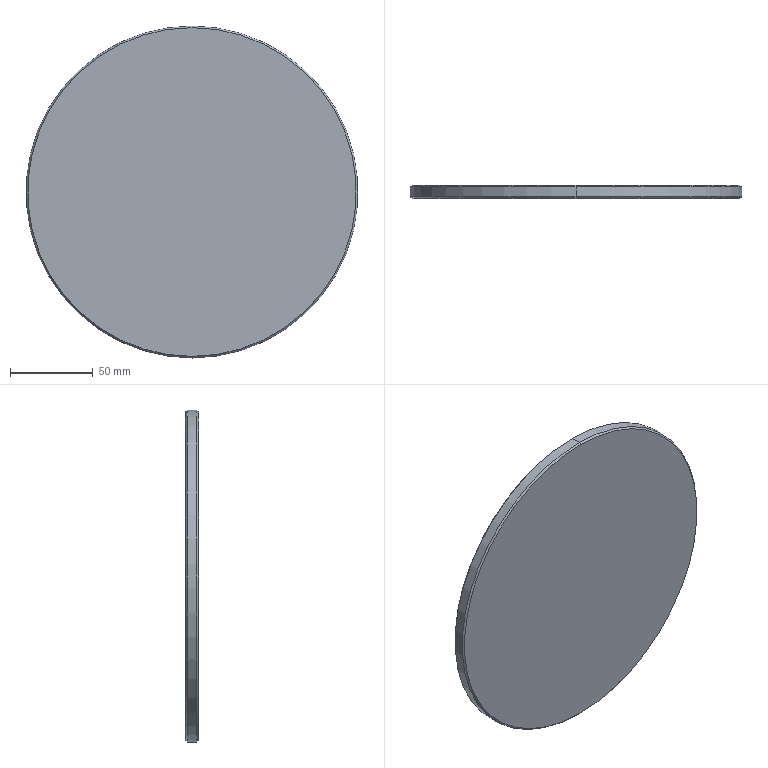Component | SolidWorks | Inline-H010-H01-001K-1 | 1 solid | 8 faces | box 200 x 8 x 200 mm | volume 250701 mm3 | cone 4 | cylinder 2 | plane 2 | commonest cylinder face diameters 200 x2
build123d program:
from build123d import *

# Parameters (mm, degrees)
SKETCH1_R           = 100
BOSS_EXTRUDE1_DEPTH = 4
CHAMFER1_SIZE       = 1


with BuildPart() as part:
    # Sketch1 → Boss-Extrude1 (new, symmetric)
    with BuildSketch(Plane.XY):
        Circle(SKETCH1_R)
    extrude(amount=BOSS_EXTRUDE1_DEPTH, both=True)

    # Chamfer1
    chamfer1_edges = [part.edges().sort_by_distance(p)[0] for p in [
        (-100, 0, -4),
        (-100, 0, 4),
    ]]
    chamfer(chamfer1_edges, length=CHAMFER1_SIZE)


solid = part.part

# Placed as in the assembly
solid = solid.moved(Location((29.082, -10.032, 139.665), (90, 0, 0)))
STEP:
#1=CARTESIAN_POINT('',(1.145,-0.2375,9.396));
#2=VERTEX_POINT('',#1);
#3=CARTESIAN_POINT('',(1.145,-0.2375,1.601));
#4=VERTEX_POINT('',#3);
#5=CARTESIAN_POINT('',(1.145,-0.2375,5.499));
#6=DIRECTION('',(-0.,1.,0.));
#7=DIRECTION('',(0.,0.,-1.));
#8=AXIS2_PLACEMENT_3D('',#5,#6,#7);
#9=CIRCLE('',#8,3.898);
#10=EDGE_CURVE('',#2,#4,#9,.T.);
#11=ORIENTED_EDGE('',*,*,#10,.F.);
#12=CARTESIAN_POINT('',(1.145,-0.2769,9.436));
#13=VERTEX_POINT('',#12);
#14=CARTESIAN_POINT('',(1.145,-0.2769,9.436));
#15=DIRECTION('',(0.,-0.7071,0.7071));
#16=VECTOR('',#15,39.37);
#17=LINE('',#14,#16);
#18=EDGE_CURVE('',#2,#13,#17,.T.);
#19=ORIENTED_EDGE('',*,*,#18,.T.);
#20=CARTESIAN_POINT('',(1.145,-0.2769,1.562));
#21=VERTEX_POINT('',#20);
#22=CARTESIAN_POINT('',(1.145,-0.2769,5.499));
#23=DIRECTION('',(0.,-1.,-0.));
#24=DIRECTION('',(0.,0.,-1.));
#25=AXIS2_PLACEMENT_3D('',#22,#23,#24);
#26=CIRCLE('',#25,3.937);
#27=EDGE_CURVE('',#21,#13,#26,.T.);
#28=ORIENTED_EDGE('',*,*,#27,.F.);
#29=CARTESIAN_POINT('',(1.145,-0.2769,1.562));
#30=DIRECTION('',(0.,-0.7071,-0.7071));
#31=VECTOR('',#30,39.37);
#32=LINE('',#29,#31);
#33=EDGE_CURVE('',#4,#21,#32,.T.);
#34=ORIENTED_EDGE('',*,*,#33,.F.);
#35=EDGE_LOOP('',(#11,#19,#28,#34));
#36=FACE_OUTER_BOUND('',#35,.T.);
#37=CARTESIAN_POINT('',(1.145,-0.2769,5.499));
#38=DIRECTION('',(0.,-1.,-0.));
#39=DIRECTION('',(0.,0.,-1.));
#40=AXIS2_PLACEMENT_3D('',#37,#38,#39);
#41=CONICAL_SURFACE('',#40,3.937,0.7854);
#42=ADVANCED_FACE('',(#36),#41,.T.);
#43=CARTESIAN_POINT('',(1.145,-0.5525,1.601));
#44=VERTEX_POINT('',#43);
#45=CARTESIAN_POINT('',(1.145,-0.5525,9.396));
#46=VERTEX_POINT('',#45);
#47=CARTESIAN_POINT('',(1.145,-0.5525,5.499));
#48=DIRECTION('',(0.,-1.,-0.));
#49=DIRECTION('',(0.,0.,-1.));
#50=AXIS2_PLACEMENT_3D('',#47,#48,#49);
#51=CIRCLE('',#50,3.898);
#52=EDGE_CURVE('',#44,#46,#51,.T.);
#53=ORIENTED_EDGE('',*,*,#52,.F.);
#54=CARTESIAN_POINT('',(1.145,-0.5131,1.562));
#55=VERTEX_POINT('',#54);
#56=CARTESIAN_POINT('',(1.145,-0.5525,1.601));
#57=DIRECTION('',(0.,0.7071,-0.7071));
#58=VECTOR('',#57,39.37);
#59=LINE('',#56,#58);
#60=EDGE_CURVE('',#44,#55,#59,.T.);
#61=ORIENTED_EDGE('',*,*,#60,.T.);
#62=CARTESIAN_POINT('',(1.145,-0.5131,9.436));
#63=VERTEX_POINT('',#62);
#64=CARTESIAN_POINT('',(1.145,-0.5131,5.499));
#65=DIRECTION('',(-0.,1.,0.));
#66=DIRECTION('',(0.,0.,-1.));
#67=AXIS2_PLACEMENT_3D('',#64,#65,#66);
#68=CIRCLE('',#67,3.937);
#69=EDGE_CURVE('',#63,#55,#68,.T.);
#70=ORIENTED_EDGE('',*,*,#69,.F.);
#71=CARTESIAN_POINT('',(1.145,-0.5525,9.396));
#72=DIRECTION('',(-0.,0.7071,0.7071));
#73=VECTOR('',#72,39.37);
#74=LINE('',#71,#73);
#75=EDGE_CURVE('',#46,#63,#74,.T.);
#76=ORIENTED_EDGE('',*,*,#75,.F.);
#77=EDGE_LOOP('',(#53,#61,#70,#76));
#78=FACE_OUTER_BOUND('',#77,.T.);
#79=CARTESIAN_POINT('',(1.145,-0.5525,5.499));
#80=DIRECTION('',(-0.,1.,0.));
#81=DIRECTION('',(0.,-0.,1.));
#82=AXIS2_PLACEMENT_3D('',#79,#80,#81);
#83=CONICAL_SURFACE('',#82,3.898,0.7854);
#84=ADVANCED_FACE('',(#78),#83,.T.);
#85=ORIENTED_EDGE('',*,*,#69,.T.);
#86=CARTESIAN_POINT('',(1.145,-0.5525,1.562));
#87=DIRECTION('',(-0.,1.,0.));
#88=VECTOR('',#87,39.37);
#89=LINE('',#86,#88);
#90=EDGE_CURVE('',#55,#21,#89,.T.);
#91=ORIENTED_EDGE('',*,*,#90,.T.);
#92=ORIENTED_EDGE('',*,*,#27,.T.);
#93=CARTESIAN_POINT('',(1.145,-0.5525,9.436));
#94=DIRECTION('',(-0.,1.,0.));
#95=VECTOR('',#94,39.37);
#96=LINE('',#93,#95);
#97=EDGE_CURVE('',#63,#13,#96,.T.);
#98=ORIENTED_EDGE('',*,*,#97,.F.);
#99=EDGE_LOOP('',(#85,#91,#92,#98));
#100=FACE_OUTER_BOUND('',#99,.T.);
#101=CARTESIAN_POINT('',(1.145,-0.5525,5.499));
#102=DIRECTION('',(-0.,1.,0.));
#103=DIRECTION('',(0.,-0.,1.));
#104=AXIS2_PLACEMENT_3D('',#101,#102,#103);
#105=CYLINDRICAL_SURFACE('',#104,3.937);
#106=ADVANCED_FACE('',(#100),#105,.T.);
#107=ORIENTED_EDGE('',*,*,#90,.F.);
#108=CARTESIAN_POINT('',(1.145,-0.5131,5.499));
#109=DIRECTION('',(-0.,1.,0.));
#110=DIRECTION('',(0.,0.,-1.));
#111=AXIS2_PLACEMENT_3D('',#108,#109,#110);
#112=CIRCLE('',#111,3.937);
#113=EDGE_CURVE('',#55,#63,#112,.T.);
#114=ORIENTED_EDGE('',*,*,#113,.T.);
#115=ORIENTED_EDGE('',*,*,#97,.T.);
#116=CARTESIAN_POINT('',(1.145,-0.2769,5.499));
#117=DIRECTION('',(0.,-1.,-0.));
#118=DIRECTION('',(0.,0.,-1.));
#119=AXIS2_PLACEMENT_3D('',#116,#117,#118);
#120=CIRCLE('',#119,3.937);
#121=EDGE_CURVE('',#13,#21,#120,.T.);
#122=ORIENTED_EDGE('',*,*,#121,.T.);
#123=EDGE_LOOP('',(#107,#114,#115,#122));
#124=FACE_OUTER_BOUND('',#123,.T.);
#125=CARTESIAN_POINT('',(1.145,-0.5525,5.499));
#126=DIRECTION('',(-0.,1.,0.));
#127=DIRECTION('',(0.,-0.,1.));
#128=AXIS2_PLACEMENT_3D('',#125,#126,#127);
#129=CYLINDRICAL_SURFACE('',#128,3.937);
#130=ADVANCED_FACE('',(#124),#129,.T.);
#131=CARTESIAN_POINT('',(1.145,-0.5525,5.499));
#132=DIRECTION('',(0.,-1.,-0.));
#133=DIRECTION('',(0.,0.,-1.));
#134=AXIS2_PLACEMENT_3D('',#131,#132,#133);
#135=CIRCLE('',#134,3.898);
#136=EDGE_CURVE('',#46,#44,#135,.T.);
#137=ORIENTED_EDGE('',*,*,#136,.T.);
#138=ORIENTED_EDGE('',*,*,#52,.T.);
#139=EDGE_LOOP('',(#137,#138));
#140=FACE_OUTER_BOUND('',#139,.T.);
#141=CARTESIAN_POINT('',(1.145,-0.5525,5.499));
#142=DIRECTION('',(0.,-1.,-0.));
#143=DIRECTION('',(0.,0.,-1.));
#144=AXIS2_PLACEMENT_3D('',#141,#142,#143);
#145=PLANE('',#144);
#146=ADVANCED_FACE('',(#140),#145,.T.);
#147=CARTESIAN_POINT('',(1.145,-0.2375,5.499));
#148=DIRECTION('',(-0.,1.,0.));
#149=DIRECTION('',(0.,0.,-1.));
#150=AXIS2_PLACEMENT_3D('',#147,#148,#149);
#151=CIRCLE('',#150,3.898);
#152=EDGE_CURVE('',#4,#2,#151,.T.);
#153=ORIENTED_EDGE('',*,*,#152,.T.);
#154=ORIENTED_EDGE('',*,*,#10,.T.);
#155=EDGE_LOOP('',(#153,#154));
#156=FACE_OUTER_BOUND('',#155,.T.);
#157=CARTESIAN_POINT('',(1.145,-0.2375,5.499));
#158=DIRECTION('',(0.,-1.,-0.));
#159=DIRECTION('',(0.,0.,-1.));
#160=AXIS2_PLACEMENT_3D('',#157,#158,#159);
#161=PLANE('',#160);
#162=ADVANCED_FACE('',(#156),#161,.F.);
#163=ORIENTED_EDGE('',*,*,#60,.F.);
#164=ORIENTED_EDGE('',*,*,#136,.F.);
#165=ORIENTED_EDGE('',*,*,#75,.T.);
#166=ORIENTED_EDGE('',*,*,#113,.F.);
#167=EDGE_LOOP('',(#163,#164,#165,#166));
#168=FACE_OUTER_BOUND('',#167,.T.);
#169=CARTESIAN_POINT('',(1.145,-0.5525,5.499));
#170=DIRECTION('',(-0.,1.,0.));
#171=DIRECTION('',(0.,-0.,1.));
#172=AXIS2_PLACEMENT_3D('',#169,#170,#171);
#173=CONICAL_SURFACE('',#172,3.898,0.7854);
#174=ADVANCED_FACE('',(#168),#173,.T.);
#175=ORIENTED_EDGE('',*,*,#18,.F.);
#176=ORIENTED_EDGE('',*,*,#152,.F.);
#177=ORIENTED_EDGE('',*,*,#33,.T.);
#178=ORIENTED_EDGE('',*,*,#121,.F.);
#179=EDGE_LOOP('',(#175,#176,#177,#178));
#180=FACE_OUTER_BOUND('',#179,.T.);
#181=CARTESIAN_POINT('',(1.145,-0.2769,5.499));
#182=DIRECTION('',(0.,-1.,-0.));
#183=DIRECTION('',(0.,0.,-1.));
#184=AXIS2_PLACEMENT_3D('',#181,#182,#183);
#185=CONICAL_SURFACE('',#184,3.937,0.7854);
#186=ADVANCED_FACE('',(#180),#185,.T.);
#187=CLOSED_SHELL('',(#42,#84,#106,#130,#146,#162,#174,#186));
#188=MANIFOLD_SOLID_BREP('',#187);
#189=CARTESIAN_POINT('',(0.,0.,0.));
#190=DIRECTION('',(0.,0.,1.));
#191=DIRECTION('',(1.,0.,0.));
#192=AXIS2_PLACEMENT_3D('',#189,#190,#191);
#193=(LENGTH_UNIT()NAMED_UNIT(*)SI_UNIT($,.METRE.));
#194=LENGTH_MEASURE_WITH_UNIT(LENGTH_MEASURE(0.0254),#193);
#195=DIMENSIONAL_EXPONENTS(1.,0.,0.,0.,0.,0.,0.);
#196=(CONVERSION_BASED_UNIT('',#194)LENGTH_UNIT()NAMED_UNIT(#195));
#197=UNCERTAINTY_MEASURE_WITH_UNIT(LENGTH_MEASURE(0.00001),#196,'','');
#198=(NAMED_UNIT(*)PLANE_ANGLE_UNIT()SI_UNIT($,.RADIAN.));
#199=(NAMED_UNIT(*)SI_UNIT($,.STERADIAN.)SOLID_ANGLE_UNIT());
#200=(GEOMETRIC_REPRESENTATION_CONTEXT(3)GLOBAL_UNCERTAINTY_ASSIGNED_CONTEXT((#197))GLOBAL_UNIT_ASSIGNED_CONTEXT((#196,#198,#199))REPRESENTATION_CONTEXT('',''));
#201=ADVANCED_BREP_SHAPE_REPRESENTATION('',(#188,#192),#200);
#202=COLOUR_RGB('',0.7922,0.8196,0.9333);
#203=FILL_AREA_STYLE_COLOUR('',#202);
#204=FILL_AREA_STYLE('',(#203));
#205=SURFACE_STYLE_FILL_AREA(#204);
#206=SURFACE_SIDE_STYLE('',(#205));
#207=SURFACE_STYLE_USAGE(.BOTH.,#206);
#208=PRESENTATION_STYLE_ASSIGNMENT((#207));
#209=STYLED_ITEM('',(#208),#188);
#210=PRESENTATION_LAYER_ASSIGNMENT('','',(#209));
#211=(LENGTH_UNIT()NAMED_UNIT(*)SI_UNIT($,.METRE.));
#212=LENGTH_MEASURE_WITH_UNIT(LENGTH_MEASURE(0.0254),#211);
#213=DIMENSIONAL_EXPONENTS(1.,0.,0.,0.,0.,0.,0.);
#214=(CONVERSION_BASED_UNIT('',#212)LENGTH_UNIT()NAMED_UNIT(#213));
#215=UNCERTAINTY_MEASURE_WITH_UNIT(LENGTH_MEASURE(0.00001),#214,'','');
#216=(NAMED_UNIT(*)PLANE_ANGLE_UNIT()SI_UNIT($,.RADIAN.));
#217=(NAMED_UNIT(*)SI_UNIT($,.STERADIAN.)SOLID_ANGLE_UNIT());
#218=(GEOMETRIC_REPRESENTATION_CONTEXT(3)GLOBAL_UNCERTAINTY_ASSIGNED_CONTEXT((#215))GLOBAL_UNIT_ASSIGNED_CONTEXT((#214,#216,#217))REPRESENTATION_CONTEXT('',''));
#219=MECHANICAL_DESIGN_GEOMETRIC_PRESENTATION_REPRESENTATION('',(#209),#218);